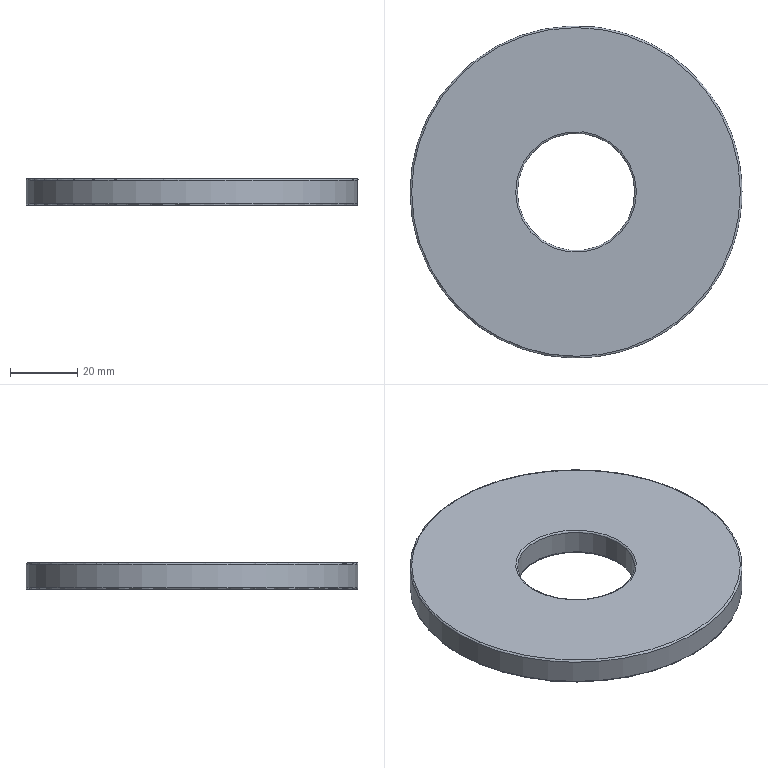Component | NX | ROUND_HOLE_WASHER | 1 solid | 8 faces | box 99 x 99 x 8 mm | volume 53839 mm3 | torus 4 | cylinder 2 | plane 2 | commonest cylinder face diameters 99 x1 35 x1
STEP:
#1=CARTESIAN_POINT('',(0.,0.,0.));
#2=DIRECTION('',(0.,0.,1.));
#3=DIRECTION('',(1.,0.,0.));
#4=AXIS2_PLACEMENT_3D('',#1,#2,#3);
#5=CARTESIAN_POINT('',(303.417,257.136,31.484));
#6=VERTEX_POINT('',#5);
#7=CARTESIAN_POINT('',(352.917,257.26,31.484));
#8=DIRECTION('',(0.,0.,1.));
#9=DIRECTION('',(-1.,-0.0025,0.));
#10=AXIS2_PLACEMENT_3D('',#7,#8,#9);
#11=CIRCLE('',#10,49.5);
#12=CARTESIAN_POINT('',(352.917,257.26,38.984));
#13=DIRECTION('',(0.,0.,-1.));
#14=DIRECTION('',(-1.,-0.0025,0.));
#15=AXIS2_PLACEMENT_3D('',#12,#13,#14);
#16=CYLINDRICAL_SURFACE('',#15,49.5);
#17=CARTESIAN_POINT('',(6.283,7.5));
#18=DIRECTION('',(-1.,0.));
#19=VECTOR('',#18,1.);
#20=LINE('',#17,#19);
#21=(GEOMETRIC_REPRESENTATION_CONTEXT(2)PARAMETRIC_REPRESENTATION_CONTEXT()REPRESENTATION_CONTEXT('',''));
#22=DEFINITIONAL_REPRESENTATION('',(#20),#21);
#23=PCURVE('',#16,#22);
#24=CARTESIAN_POINT('',(352.917,257.26,31.484));
#25=DIRECTION('',(0.,0.,-1.));
#26=DIRECTION('',(-1.,-0.0025,0.));
#27=AXIS2_PLACEMENT_3D('',#24,#25,#26);
#28=TOROIDAL_SURFACE('',#27,49.,0.5);
#29=CARTESIAN_POINT('',(6.283,6.283));
#30=DIRECTION('',(-1.,0.));
#31=VECTOR('',#30,1.);
#32=LINE('',#29,#31);
#33=(GEOMETRIC_REPRESENTATION_CONTEXT(2)PARAMETRIC_REPRESENTATION_CONTEXT()REPRESENTATION_CONTEXT('',''));
#34=DEFINITIONAL_REPRESENTATION('',(#32),#33);
#35=PCURVE('',#28,#34);
#36=SURFACE_CURVE('',#11,(#23,#35),.PCURVE_S1.);
#37=EDGE_CURVE('',#6,#6,#36,.T.);
#38=ORIENTED_EDGE('',*,*,#37,.T.);
#39=CARTESIAN_POINT('',(303.417,257.136,38.484));
#40=VERTEX_POINT('',#39);
#41=CARTESIAN_POINT('',(303.417,257.136,38.484));
#42=CARTESIAN_POINT('',(303.417,257.136,31.484));
#43=B_SPLINE_CURVE_WITH_KNOTS('',1,(#41,#42),.UNSPECIFIED.,.F.,.F.,(2,2),(0.5,7.5),.PIECEWISE_BEZIER_KNOTS.);
#44=CARTESIAN_POINT('',(0.,0.));
#45=DIRECTION('',(0.,1.));
#46=VECTOR('',#45,1.);
#47=LINE('',#44,#46);
#48=(GEOMETRIC_REPRESENTATION_CONTEXT(2)PARAMETRIC_REPRESENTATION_CONTEXT()REPRESENTATION_CONTEXT('',''));
#49=DEFINITIONAL_REPRESENTATION('',(#47),#48);
#50=PCURVE('',#16,#49);
#51=CARTESIAN_POINT('',(6.283,0.));
#52=DIRECTION('',(0.,1.));
#53=VECTOR('',#52,1.);
#54=LINE('',#51,#53);
#55=(GEOMETRIC_REPRESENTATION_CONTEXT(2)PARAMETRIC_REPRESENTATION_CONTEXT()REPRESENTATION_CONTEXT('',''));
#56=DEFINITIONAL_REPRESENTATION('',(#54),#55);
#57=PCURVE('',#16,#56);
#58=SEAM_CURVE('',#43,(#50,#57),.PCURVE_S1.);
#59=EDGE_CURVE('',#40,#6,#58,.T.);
#60=ORIENTED_EDGE('',*,*,#59,.F.);
#61=CARTESIAN_POINT('',(352.917,257.26,38.484));
#62=DIRECTION('',(0.,0.,-1.));
#63=DIRECTION('',(-1.,-0.0025,0.));
#64=AXIS2_PLACEMENT_3D('',#61,#62,#63);
#65=CIRCLE('',#64,49.5);
#66=CARTESIAN_POINT('',(0.,0.5));
#67=DIRECTION('',(1.,0.));
#68=VECTOR('',#67,1.);
#69=LINE('',#66,#68);
#70=(GEOMETRIC_REPRESENTATION_CONTEXT(2)PARAMETRIC_REPRESENTATION_CONTEXT()REPRESENTATION_CONTEXT('',''));
#71=DEFINITIONAL_REPRESENTATION('',(#69),#70);
#72=PCURVE('',#16,#71);
#73=CARTESIAN_POINT('',(352.917,257.26,38.484));
#74=DIRECTION('',(0.,0.,-1.));
#75=DIRECTION('',(-1.,-0.0025,0.));
#76=AXIS2_PLACEMENT_3D('',#73,#74,#75);
#77=TOROIDAL_SURFACE('',#76,49.,0.5);
#78=CARTESIAN_POINT('',(0.,6.283));
#79=DIRECTION('',(1.,0.));
#80=VECTOR('',#79,1.);
#81=LINE('',#78,#80);
#82=(GEOMETRIC_REPRESENTATION_CONTEXT(2)PARAMETRIC_REPRESENTATION_CONTEXT()REPRESENTATION_CONTEXT('',''));
#83=DEFINITIONAL_REPRESENTATION('',(#81),#82);
#84=PCURVE('',#77,#83);
#85=SURFACE_CURVE('',#65,(#72,#84),.PCURVE_S1.);
#86=EDGE_CURVE('',#40,#40,#85,.T.);
#87=ORIENTED_EDGE('',*,*,#86,.T.);
#88=ORIENTED_EDGE('',*,*,#59,.T.);
#89=EDGE_LOOP('',(#38,#60,#87,#88));
#90=FACE_BOUND('',#89,.T.);
#91=ADVANCED_FACE('',(#90),#16,.T.);
#92=CARTESIAN_POINT('',(335.417,257.216,31.484));
#93=VERTEX_POINT('',#92);
#94=CARTESIAN_POINT('',(352.917,257.26,31.484));
#95=DIRECTION('',(0.,0.,-1.));
#96=DIRECTION('',(-1.,-0.0025,0.));
#97=AXIS2_PLACEMENT_3D('',#94,#95,#96);
#98=CIRCLE('',#97,17.5);
#99=CARTESIAN_POINT('',(352.917,257.26,38.984));
#100=DIRECTION('',(0.,0.,-1.));
#101=DIRECTION('',(-1.,-0.0025,0.));
#102=AXIS2_PLACEMENT_3D('',#99,#100,#101);
#103=CYLINDRICAL_SURFACE('',#102,17.5);
#104=CARTESIAN_POINT('',(0.,7.5));
#105=DIRECTION('',(1.,0.));
#106=VECTOR('',#105,1.);
#107=LINE('',#104,#106);
#108=(GEOMETRIC_REPRESENTATION_CONTEXT(2)PARAMETRIC_REPRESENTATION_CONTEXT()REPRESENTATION_CONTEXT('',''));
#109=DEFINITIONAL_REPRESENTATION('',(#107),#108);
#110=PCURVE('',#103,#109);
#111=CARTESIAN_POINT('',(352.917,257.26,31.484));
#112=DIRECTION('',(0.,0.,-1.));
#113=DIRECTION('',(-1.,-0.0025,0.));
#114=AXIS2_PLACEMENT_3D('',#111,#112,#113);
#115=TOROIDAL_SURFACE('',#114,18.,0.5);
#116=CARTESIAN_POINT('',(0.,9.425));
#117=DIRECTION('',(1.,0.));
#118=VECTOR('',#117,1.);
#119=LINE('',#116,#118);
#120=(GEOMETRIC_REPRESENTATION_CONTEXT(2)PARAMETRIC_REPRESENTATION_CONTEXT()REPRESENTATION_CONTEXT('',''));
#121=DEFINITIONAL_REPRESENTATION('',(#119),#120);
#122=PCURVE('',#115,#121);
#123=SURFACE_CURVE('',#98,(#110,#122),.PCURVE_S1.);
#124=EDGE_CURVE('',#93,#93,#123,.T.);
#125=ORIENTED_EDGE('',*,*,#124,.F.);
#126=CARTESIAN_POINT('',(335.417,257.216,38.484));
#127=VERTEX_POINT('',#126);
#128=CARTESIAN_POINT('',(335.417,257.216,38.484));
#129=CARTESIAN_POINT('',(335.417,257.216,31.484));
#130=B_SPLINE_CURVE_WITH_KNOTS('',1,(#128,#129),.UNSPECIFIED.,.F.,.F.,(2,2),(0.5,7.5),.PIECEWISE_BEZIER_KNOTS.);
#131=CARTESIAN_POINT('',(0.,0.));
#132=DIRECTION('',(0.,1.));
#133=VECTOR('',#132,1.);
#134=LINE('',#131,#133);
#135=(GEOMETRIC_REPRESENTATION_CONTEXT(2)PARAMETRIC_REPRESENTATION_CONTEXT()REPRESENTATION_CONTEXT('',''));
#136=DEFINITIONAL_REPRESENTATION('',(#134),#135);
#137=PCURVE('',#103,#136);
#138=CARTESIAN_POINT('',(6.283,0.));
#139=DIRECTION('',(0.,1.));
#140=VECTOR('',#139,1.);
#141=LINE('',#138,#140);
#142=(GEOMETRIC_REPRESENTATION_CONTEXT(2)PARAMETRIC_REPRESENTATION_CONTEXT()REPRESENTATION_CONTEXT('',''));
#143=DEFINITIONAL_REPRESENTATION('',(#141),#142);
#144=PCURVE('',#103,#143);
#145=SEAM_CURVE('',#130,(#137,#144),.PCURVE_S1.);
#146=EDGE_CURVE('',#127,#93,#145,.T.);
#147=ORIENTED_EDGE('',*,*,#146,.F.);
#148=CARTESIAN_POINT('',(352.917,257.26,38.484));
#149=DIRECTION('',(0.,0.,1.));
#150=DIRECTION('',(-1.,-0.0025,0.));
#151=AXIS2_PLACEMENT_3D('',#148,#149,#150);
#152=CIRCLE('',#151,17.5);
#153=CARTESIAN_POINT('',(6.283,0.5));
#154=DIRECTION('',(-1.,0.));
#155=VECTOR('',#154,1.);
#156=LINE('',#153,#155);
#157=(GEOMETRIC_REPRESENTATION_CONTEXT(2)PARAMETRIC_REPRESENTATION_CONTEXT()REPRESENTATION_CONTEXT('',''));
#158=DEFINITIONAL_REPRESENTATION('',(#156),#157);
#159=PCURVE('',#103,#158);
#160=CARTESIAN_POINT('',(352.917,257.26,38.484));
#161=DIRECTION('',(0.,0.,-1.));
#162=DIRECTION('',(-1.,-0.0025,0.));
#163=AXIS2_PLACEMENT_3D('',#160,#161,#162);
#164=TOROIDAL_SURFACE('',#163,18.,0.5);
#165=CARTESIAN_POINT('',(6.283,3.142));
#166=DIRECTION('',(-1.,0.));
#167=VECTOR('',#166,1.);
#168=LINE('',#165,#167);
#169=(GEOMETRIC_REPRESENTATION_CONTEXT(2)PARAMETRIC_REPRESENTATION_CONTEXT()REPRESENTATION_CONTEXT('',''));
#170=DEFINITIONAL_REPRESENTATION('',(#168),#169);
#171=PCURVE('',#164,#170);
#172=SURFACE_CURVE('',#152,(#159,#171),.PCURVE_S1.);
#173=EDGE_CURVE('',#127,#127,#172,.T.);
#174=ORIENTED_EDGE('',*,*,#173,.F.);
#175=ORIENTED_EDGE('',*,*,#146,.T.);
#176=EDGE_LOOP('',(#125,#147,#174,#175));
#177=FACE_BOUND('',#176,.F.);
#178=ADVANCED_FACE('',(#177),#103,.F.);
#179=CARTESIAN_POINT('',(334.917,257.215,38.984));
#180=VERTEX_POINT('',#179);
#181=CARTESIAN_POINT('',(352.917,257.26,38.984));
#182=DIRECTION('',(0.,0.,-1.));
#183=DIRECTION('',(-1.,-0.0025,0.));
#184=AXIS2_PLACEMENT_3D('',#181,#182,#183);
#185=CIRCLE('',#184,18.);
#186=CARTESIAN_POINT('',(352.917,257.26,38.984));
#187=DIRECTION('',(0.,0.,-1.));
#188=DIRECTION('',(-1.,-0.0025,0.));
#189=AXIS2_PLACEMENT_3D('',#186,#187,#188);
#190=PLANE('',#189);
#191=CARTESIAN_POINT('',(0.,0.));
#192=DIRECTION('',(1.,-0.));
#193=AXIS2_PLACEMENT_2D('',#191,#192);
#194=CIRCLE('',#193,18.);
#195=(GEOMETRIC_REPRESENTATION_CONTEXT(2)PARAMETRIC_REPRESENTATION_CONTEXT()REPRESENTATION_CONTEXT('',''));
#196=DEFINITIONAL_REPRESENTATION('',(#194),#195);
#197=PCURVE('',#190,#196);
#198=CARTESIAN_POINT('',(0.,4.712));
#199=DIRECTION('',(1.,0.));
#200=VECTOR('',#199,1.);
#201=LINE('',#198,#200);
#202=(GEOMETRIC_REPRESENTATION_CONTEXT(2)PARAMETRIC_REPRESENTATION_CONTEXT()REPRESENTATION_CONTEXT('',''));
#203=DEFINITIONAL_REPRESENTATION('',(#201),#202);
#204=PCURVE('',#164,#203);
#205=SURFACE_CURVE('',#185,(#197,#204),.PCURVE_S1.);
#206=EDGE_CURVE('',#180,#180,#205,.T.);
#207=ORIENTED_EDGE('',*,*,#206,.T.);
#208=EDGE_LOOP('',(#207));
#209=FACE_BOUND('',#208,.T.);
#210=CARTESIAN_POINT('',(303.917,257.137,38.984));
#211=VERTEX_POINT('',#210);
#212=CARTESIAN_POINT('',(352.917,257.26,38.984));
#213=DIRECTION('',(0.,0.,1.));
#214=DIRECTION('',(-1.,-0.0025,0.));
#215=AXIS2_PLACEMENT_3D('',#212,#213,#214);
#216=CIRCLE('',#215,49.);
#217=CARTESIAN_POINT('',(49.,-0.));
#218=CARTESIAN_POINT('',(49.,-84.87));
#219=CARTESIAN_POINT('',(-24.5,-42.435));
#220=CARTESIAN_POINT('',(-98.,0.));
#221=CARTESIAN_POINT('',(-24.5,42.435));
#222=CARTESIAN_POINT('',(49.,84.87));
#223=CARTESIAN_POINT('',(49.,-0.));
#224=(BOUNDED_CURVE()B_SPLINE_CURVE(2,(#217,#218,#219,#220,#221,#222,#223),.UNSPECIFIED.,.T.,.F.)B_SPLINE_CURVE_WITH_KNOTS((1,2,2,2,2,1),(-2.094,0.,2.094,4.189,6.283,8.378),.UNSPECIFIED.)CURVE()GEOMETRIC_REPRESENTATION_ITEM()RATIONAL_B_SPLINE_CURVE((1.,0.5,1.,0.5,1.,0.5,1.))REPRESENTATION_ITEM(''));
#225=(GEOMETRIC_REPRESENTATION_CONTEXT(2)PARAMETRIC_REPRESENTATION_CONTEXT()REPRESENTATION_CONTEXT('',''));
#226=DEFINITIONAL_REPRESENTATION('',(#224),#225);
#227=PCURVE('',#190,#226);
#228=CARTESIAN_POINT('',(6.283,4.712));
#229=DIRECTION('',(-1.,0.));
#230=VECTOR('',#229,1.);
#231=LINE('',#228,#230);
#232=(GEOMETRIC_REPRESENTATION_CONTEXT(2)PARAMETRIC_REPRESENTATION_CONTEXT()REPRESENTATION_CONTEXT('',''));
#233=DEFINITIONAL_REPRESENTATION('',(#231),#232);
#234=PCURVE('',#77,#233);
#235=SURFACE_CURVE('',#216,(#227,#234),.PCURVE_S1.);
#236=EDGE_CURVE('',#211,#211,#235,.T.);
#237=ORIENTED_EDGE('',*,*,#236,.T.);
#238=EDGE_LOOP('',(#237));
#239=FACE_BOUND('',#238,.T.);
#240=ADVANCED_FACE('',(#209,#239),#190,.F.);
#241=CARTESIAN_POINT('',(334.917,257.215,30.984));
#242=VERTEX_POINT('',#241);
#243=CARTESIAN_POINT('',(352.917,257.26,30.984));
#244=DIRECTION('',(0.,0.,1.));
#245=DIRECTION('',(-1.,-0.0025,0.));
#246=AXIS2_PLACEMENT_3D('',#243,#244,#245);
#247=CIRCLE('',#246,18.);
#248=CARTESIAN_POINT('',(352.917,257.26,30.984));
#249=DIRECTION('',(0.,0.,-1.));
#250=DIRECTION('',(-1.,-0.0025,0.));
#251=AXIS2_PLACEMENT_3D('',#248,#249,#250);
#252=PLANE('',#251);
#253=CARTESIAN_POINT('',(18.,-0.));
#254=CARTESIAN_POINT('',(18.,-31.177));
#255=CARTESIAN_POINT('',(-9.,-15.588));
#256=CARTESIAN_POINT('',(-36.,0.));
#257=CARTESIAN_POINT('',(-9.,15.588));
#258=CARTESIAN_POINT('',(18.,31.177));
#259=CARTESIAN_POINT('',(18.,-0.));
#260=(BOUNDED_CURVE()B_SPLINE_CURVE(2,(#253,#254,#255,#256,#257,#258,#259),.UNSPECIFIED.,.T.,.F.)B_SPLINE_CURVE_WITH_KNOTS((1,2,2,2,2,1),(-2.094,0.,2.094,4.189,6.283,8.378),.UNSPECIFIED.)CURVE()GEOMETRIC_REPRESENTATION_ITEM()RATIONAL_B_SPLINE_CURVE((1.,0.5,1.,0.5,1.,0.5,1.))REPRESENTATION_ITEM(''));
#261=(GEOMETRIC_REPRESENTATION_CONTEXT(2)PARAMETRIC_REPRESENTATION_CONTEXT()REPRESENTATION_CONTEXT('',''));
#262=DEFINITIONAL_REPRESENTATION('',(#260),#261);
#263=PCURVE('',#252,#262);
#264=CARTESIAN_POINT('',(6.283,7.854));
#265=DIRECTION('',(-1.,0.));
#266=VECTOR('',#265,1.);
#267=LINE('',#264,#266);
#268=(GEOMETRIC_REPRESENTATION_CONTEXT(2)PARAMETRIC_REPRESENTATION_CONTEXT()REPRESENTATION_CONTEXT('',''));
#269=DEFINITIONAL_REPRESENTATION('',(#267),#268);
#270=PCURVE('',#115,#269);
#271=SURFACE_CURVE('',#247,(#263,#270),.PCURVE_S1.);
#272=EDGE_CURVE('',#242,#242,#271,.T.);
#273=ORIENTED_EDGE('',*,*,#272,.T.);
#274=EDGE_LOOP('',(#273));
#275=FACE_BOUND('',#274,.T.);
#276=CARTESIAN_POINT('',(303.917,257.137,30.984));
#277=VERTEX_POINT('',#276);
#278=CARTESIAN_POINT('',(352.917,257.26,30.984));
#279=DIRECTION('',(0.,0.,-1.));
#280=DIRECTION('',(-1.,-0.0025,0.));
#281=AXIS2_PLACEMENT_3D('',#278,#279,#280);
#282=CIRCLE('',#281,49.);
#283=CARTESIAN_POINT('',(0.,0.));
#284=DIRECTION('',(1.,-0.));
#285=AXIS2_PLACEMENT_2D('',#283,#284);
#286=CIRCLE('',#285,49.);
#287=(GEOMETRIC_REPRESENTATION_CONTEXT(2)PARAMETRIC_REPRESENTATION_CONTEXT()REPRESENTATION_CONTEXT('',''));
#288=DEFINITIONAL_REPRESENTATION('',(#286),#287);
#289=PCURVE('',#252,#288);
#290=CARTESIAN_POINT('',(0.,7.854));
#291=DIRECTION('',(1.,0.));
#292=VECTOR('',#291,1.);
#293=LINE('',#290,#292);
#294=(GEOMETRIC_REPRESENTATION_CONTEXT(2)PARAMETRIC_REPRESENTATION_CONTEXT()REPRESENTATION_CONTEXT('',''));
#295=DEFINITIONAL_REPRESENTATION('',(#293),#294);
#296=PCURVE('',#28,#295);
#297=SURFACE_CURVE('',#282,(#289,#296),.PCURVE_S1.);
#298=EDGE_CURVE('',#277,#277,#297,.T.);
#299=ORIENTED_EDGE('',*,*,#298,.T.);
#300=EDGE_LOOP('',(#299));
#301=FACE_BOUND('',#300,.T.);
#302=ADVANCED_FACE('',(#275,#301),#252,.T.);
#303=ORIENTED_EDGE('',*,*,#37,.F.);
#304=CARTESIAN_POINT('',(303.417,257.136,31.484));
#305=CARTESIAN_POINT('',(303.417,257.136,31.35));
#306=CARTESIAN_POINT('',(303.459,257.136,31.22));
#307=CARTESIAN_POINT('',(303.541,257.136,31.108));
#308=CARTESIAN_POINT('',(303.653,257.136,31.026));
#309=CARTESIAN_POINT('',(303.783,257.137,30.984));
#310=CARTESIAN_POINT('',(303.917,257.137,30.984));
#311=(BOUNDED_CURVE()B_SPLINE_CURVE(6,(#304,#305,#306,#307,#308,#309,#310),.UNSPECIFIED.,.F.,.F.)B_SPLINE_CURVE_WITH_KNOTS((7,7),(0.,1.571),.PIECEWISE_BEZIER_KNOTS.)CURVE()GEOMETRIC_REPRESENTATION_ITEM()RATIONAL_B_SPLINE_CURVE((1.031,1.01,0.9979,0.994,0.9979,1.01,1.031))REPRESENTATION_ITEM(''));
#312=CARTESIAN_POINT('',(6.283,6.283));
#313=DIRECTION('',(0.,1.));
#314=VECTOR('',#313,1.);
#315=LINE('',#312,#314);
#316=(GEOMETRIC_REPRESENTATION_CONTEXT(2)PARAMETRIC_REPRESENTATION_CONTEXT()REPRESENTATION_CONTEXT('',''));
#317=DEFINITIONAL_REPRESENTATION('',(#315),#316);
#318=PCURVE('',#28,#317);
#319=CARTESIAN_POINT('',(0.,6.283));
#320=DIRECTION('',(0.,1.));
#321=VECTOR('',#320,1.);
#322=LINE('',#319,#321);
#323=(GEOMETRIC_REPRESENTATION_CONTEXT(2)PARAMETRIC_REPRESENTATION_CONTEXT()REPRESENTATION_CONTEXT('',''));
#324=DEFINITIONAL_REPRESENTATION('',(#322),#323);
#325=PCURVE('',#28,#324);
#326=SEAM_CURVE('',#311,(#318,#325),.PCURVE_S1.);
#327=EDGE_CURVE('',#6,#277,#326,.T.);
#328=ORIENTED_EDGE('',*,*,#327,.T.);
#329=ORIENTED_EDGE('',*,*,#298,.F.);
#330=ORIENTED_EDGE('',*,*,#327,.F.);
#331=EDGE_LOOP('',(#303,#328,#329,#330));
#332=FACE_BOUND('',#331,.T.);
#333=ADVANCED_FACE('',(#332),#28,.T.);
#334=ORIENTED_EDGE('',*,*,#236,.F.);
#335=CARTESIAN_POINT('',(303.917,257.137,38.984));
#336=CARTESIAN_POINT('',(303.783,257.137,38.984));
#337=CARTESIAN_POINT('',(303.653,257.136,38.941));
#338=CARTESIAN_POINT('',(303.541,257.136,38.86));
#339=CARTESIAN_POINT('',(303.459,257.136,38.748));
#340=CARTESIAN_POINT('',(303.417,257.136,38.617));
#341=CARTESIAN_POINT('',(303.417,257.136,38.484));
#342=(BOUNDED_CURVE()B_SPLINE_CURVE(6,(#335,#336,#337,#338,#339,#340,#341),.UNSPECIFIED.,.F.,.F.)B_SPLINE_CURVE_WITH_KNOTS((7,7),(4.712,6.283),.PIECEWISE_BEZIER_KNOTS.)CURVE()GEOMETRIC_REPRESENTATION_ITEM()RATIONAL_B_SPLINE_CURVE((1.031,1.01,0.9979,0.994,0.9979,1.01,1.031))REPRESENTATION_ITEM(''));
#343=CARTESIAN_POINT('',(6.283,0.));
#344=DIRECTION('',(0.,1.));
#345=VECTOR('',#344,1.);
#346=LINE('',#343,#345);
#347=(GEOMETRIC_REPRESENTATION_CONTEXT(2)PARAMETRIC_REPRESENTATION_CONTEXT()REPRESENTATION_CONTEXT('',''));
#348=DEFINITIONAL_REPRESENTATION('',(#346),#347);
#349=PCURVE('',#77,#348);
#350=CARTESIAN_POINT('',(0.,0.));
#351=DIRECTION('',(0.,1.));
#352=VECTOR('',#351,1.);
#353=LINE('',#350,#352);
#354=(GEOMETRIC_REPRESENTATION_CONTEXT(2)PARAMETRIC_REPRESENTATION_CONTEXT()REPRESENTATION_CONTEXT('',''));
#355=DEFINITIONAL_REPRESENTATION('',(#353),#354);
#356=PCURVE('',#77,#355);
#357=SEAM_CURVE('',#342,(#349,#356),.PCURVE_S1.);
#358=EDGE_CURVE('',#211,#40,#357,.T.);
#359=ORIENTED_EDGE('',*,*,#358,.T.);
#360=ORIENTED_EDGE('',*,*,#86,.F.);
#361=ORIENTED_EDGE('',*,*,#358,.F.);
#362=EDGE_LOOP('',(#334,#359,#360,#361));
#363=FACE_BOUND('',#362,.T.);
#364=ADVANCED_FACE('',(#363),#77,.T.);
#365=ORIENTED_EDGE('',*,*,#124,.F.);
#366=CARTESIAN_POINT('',(334.917,257.215,30.984));
#367=CARTESIAN_POINT('',(335.051,257.215,30.984));
#368=CARTESIAN_POINT('',(335.181,257.215,31.026));
#369=CARTESIAN_POINT('',(335.293,257.216,31.108));
#370=CARTESIAN_POINT('',(335.374,257.216,31.22));
#371=CARTESIAN_POINT('',(335.417,257.216,31.35));
#372=CARTESIAN_POINT('',(335.417,257.216,31.484));
#373=(BOUNDED_CURVE()B_SPLINE_CURVE(6,(#366,#367,#368,#369,#370,#371,#372),.UNSPECIFIED.,.F.,.F.)B_SPLINE_CURVE_WITH_KNOTS((7,7),(1.571,3.142),.PIECEWISE_BEZIER_KNOTS.)CURVE()GEOMETRIC_REPRESENTATION_ITEM()RATIONAL_B_SPLINE_CURVE((1.031,1.01,0.9979,0.994,0.9979,1.01,1.031))REPRESENTATION_ITEM(''));
#374=CARTESIAN_POINT('',(0.,6.283));
#375=DIRECTION('',(0.,1.));
#376=VECTOR('',#375,1.);
#377=LINE('',#374,#376);
#378=(GEOMETRIC_REPRESENTATION_CONTEXT(2)PARAMETRIC_REPRESENTATION_CONTEXT()REPRESENTATION_CONTEXT('',''));
#379=DEFINITIONAL_REPRESENTATION('',(#377),#378);
#380=PCURVE('',#115,#379);
#381=CARTESIAN_POINT('',(6.283,6.283));
#382=DIRECTION('',(0.,1.));
#383=VECTOR('',#382,1.);
#384=LINE('',#381,#383);
#385=(GEOMETRIC_REPRESENTATION_CONTEXT(2)PARAMETRIC_REPRESENTATION_CONTEXT()REPRESENTATION_CONTEXT('',''));
#386=DEFINITIONAL_REPRESENTATION('',(#384),#385);
#387=PCURVE('',#115,#386);
#388=SEAM_CURVE('',#373,(#380,#387),.PCURVE_S1.);
#389=EDGE_CURVE('',#242,#93,#388,.T.);
#390=ORIENTED_EDGE('',*,*,#389,.F.);
#391=ORIENTED_EDGE('',*,*,#272,.F.);
#392=ORIENTED_EDGE('',*,*,#389,.T.);
#393=EDGE_LOOP('',(#365,#390,#391,#392));
#394=FACE_BOUND('',#393,.T.);
#395=ADVANCED_FACE('',(#394),#115,.T.);
#396=ORIENTED_EDGE('',*,*,#206,.F.);
#397=CARTESIAN_POINT('',(335.417,257.216,38.484));
#398=CARTESIAN_POINT('',(335.417,257.216,38.617));
#399=CARTESIAN_POINT('',(335.374,257.216,38.748));
#400=CARTESIAN_POINT('',(335.293,257.216,38.86));
#401=CARTESIAN_POINT('',(335.181,257.215,38.941));
#402=CARTESIAN_POINT('',(335.051,257.215,38.984));
#403=CARTESIAN_POINT('',(334.917,257.215,38.984));
#404=(BOUNDED_CURVE()B_SPLINE_CURVE(6,(#397,#398,#399,#400,#401,#402,#403),.UNSPECIFIED.,.F.,.F.)B_SPLINE_CURVE_WITH_KNOTS((7,7),(3.142,4.712),.PIECEWISE_BEZIER_KNOTS.)CURVE()GEOMETRIC_REPRESENTATION_ITEM()RATIONAL_B_SPLINE_CURVE((1.031,1.01,0.9979,0.994,0.9979,1.01,1.031))REPRESENTATION_ITEM(''));
#405=CARTESIAN_POINT('',(0.,0.));
#406=DIRECTION('',(0.,1.));
#407=VECTOR('',#406,1.);
#408=LINE('',#405,#407);
#409=(GEOMETRIC_REPRESENTATION_CONTEXT(2)PARAMETRIC_REPRESENTATION_CONTEXT()REPRESENTATION_CONTEXT('',''));
#410=DEFINITIONAL_REPRESENTATION('',(#408),#409);
#411=PCURVE('',#164,#410);
#412=CARTESIAN_POINT('',(6.283,0.));
#413=DIRECTION('',(0.,1.));
#414=VECTOR('',#413,1.);
#415=LINE('',#412,#414);
#416=(GEOMETRIC_REPRESENTATION_CONTEXT(2)PARAMETRIC_REPRESENTATION_CONTEXT()REPRESENTATION_CONTEXT('',''));
#417=DEFINITIONAL_REPRESENTATION('',(#415),#416);
#418=PCURVE('',#164,#417);
#419=SEAM_CURVE('',#404,(#411,#418),.PCURVE_S1.);
#420=EDGE_CURVE('',#127,#180,#419,.T.);
#421=ORIENTED_EDGE('',*,*,#420,.F.);
#422=ORIENTED_EDGE('',*,*,#173,.F.);
#423=ORIENTED_EDGE('',*,*,#420,.T.);
#424=EDGE_LOOP('',(#396,#421,#422,#423));
#425=FACE_BOUND('',#424,.T.);
#426=ADVANCED_FACE('',(#425),#164,.T.);
#427=CLOSED_SHELL('',(#91,#178,#240,#302,#333,#364,#395,#426));
#428=MANIFOLD_SOLID_BREP('',#427);
#429=(LENGTH_UNIT()NAMED_UNIT(*)SI_UNIT(.MILLI.,.METRE.));
#430=UNCERTAINTY_MEASURE_WITH_UNIT(LENGTH_MEASURE(0.00001),#429,'','');
#431=(NAMED_UNIT(*)PLANE_ANGLE_UNIT()SI_UNIT($,.RADIAN.));
#432=(NAMED_UNIT(*)SI_UNIT($,.STERADIAN.)SOLID_ANGLE_UNIT());
#433=(GEOMETRIC_REPRESENTATION_CONTEXT(3)GLOBAL_UNCERTAINTY_ASSIGNED_CONTEXT((#430))GLOBAL_UNIT_ASSIGNED_CONTEXT((#429,#431,#432))REPRESENTATION_CONTEXT('',''));
#434=ADVANCED_BREP_SHAPE_REPRESENTATION('',(#4,#428),#433);